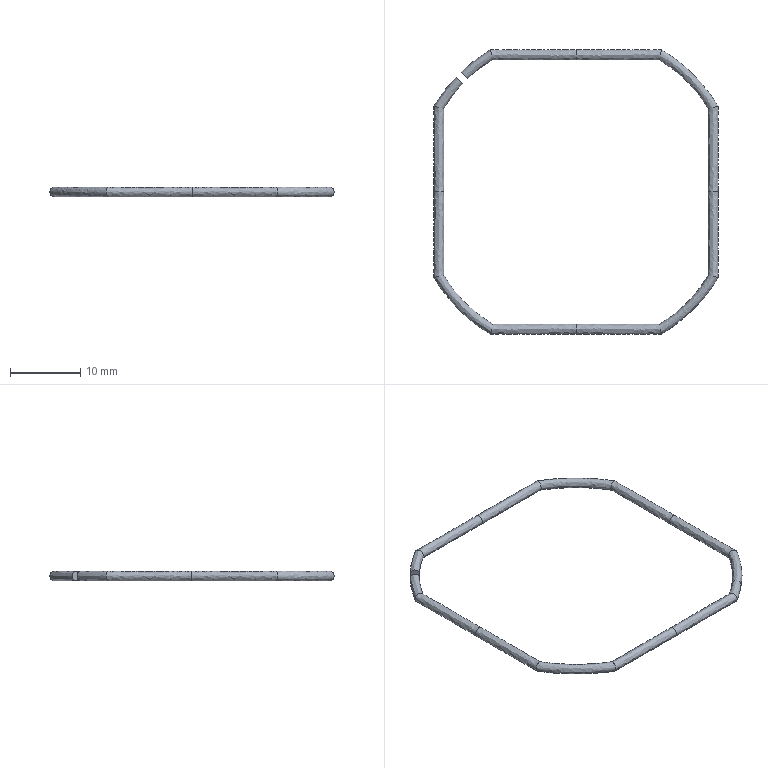Component | NX | STEEL_WIRE | 1 solid | 15 faces | volume 210 mm3 | spline 13 | plane 2